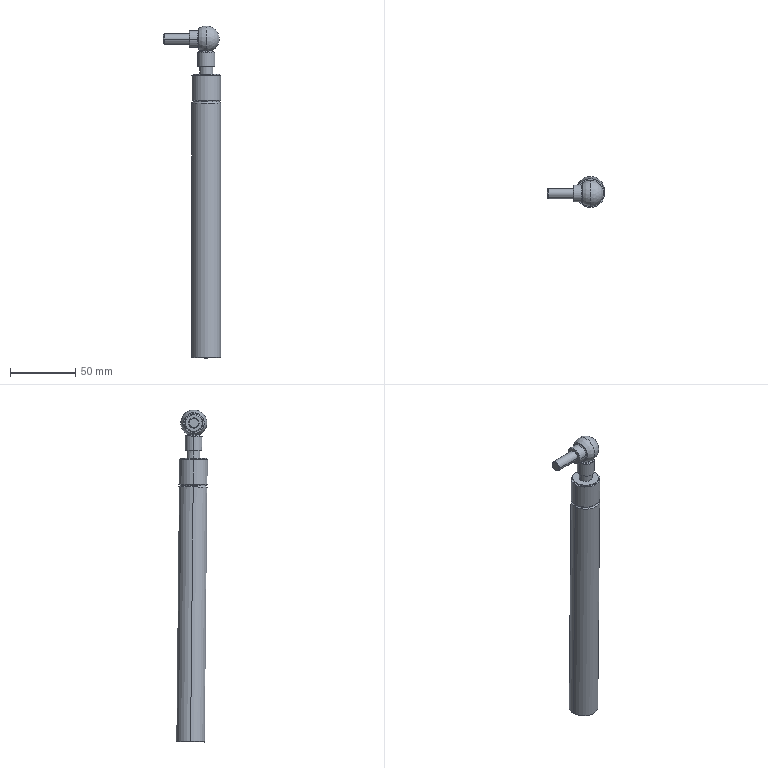Component | SolidWorks | GasSpringA-1 | 1 solid | 45 faces | box 44 x 24.24 x 255.09 mm | volume 50816 mm3 | cylinder 16 | cone 10 | plane 9 | torus 8 | sphere 2 | commonest cylinder face diameters 13 x4 22 x4 17 x2 8 x2 10 x2 20 x2
build123d program:
from build123d import *

# Parameters (mm, degrees)
SKETCH4_W           = 10.702
SKETCH4_H           = 20.307
CUT_EXTRUDE1_DEPTH  = 25
SKETCH5_R           = 6.5
BOSS_EXTRUDE1_DEPTH = 7
SKETCH6_R           = 4
BOSS_EXTRUDE2_DEPTH = 20
CHAMFER1_SIZE       = 0.5
CHAMFER2_SIZE       = 0.5
CHAMFER3_SIZE       = 0.2
SKETCH7_R           = 8.5
CUT_EXTRUDE2_DEPTH  = 600
FILLET1_R           = 1
SKETCH8_W           = 40.588
SKETCH8_H           = 852
CUT_EXTRUDE3_DEPTH  = 25
CHAMFER4_SIZE       = 0.5


with BuildPart() as part:
    # Sketch1 → Revolve1 (revolve)
    with BuildSketch(Plane.XY, mode=Mode.PRIVATE) as revolve1_sk:
        with BuildLine():
            Line((0, 0), (0, -680.998))
            ThreePointArc((0, -680.998), (-9.645, -673.639), (-5.095, -662.393))
            ThreePointArc((-5.095, -662.393), (-4.754, -661.55), (-5.477, -660.998))
            Line((-5.477, -660.998), (-6.5, -660.998))
            Line((-6.5, -660.998), (-6.5, -649.998))
            Line((-6.5, -649.998), (-5, -649.998))
            Line((-5, -649.998), (-5, -643.874))
            Line((-5, -643.874), (-10, -643.874))
            Line((-10, -643.874), (-10, -642.874))
            Line((-10, -642.874), (-11, -642.874))
            Line((-11, -642.874), (-11, -623.874))
            ThreePointArc((-11, -623.874), (-10, -622.874), (-11, -621.874))
            Line((-11, -621.874), (-11, 0))
            Line((-11, 0), (0, 0))
        make_face()
    revolve(revolve1_sk.sketch.rotate(Axis((0, 84.521, 0), (0, -1, 0)), 270), axis=Axis((0, 84.521, 0), (0, -1, 0)))

    # Sketch4 → Cut-Extrude1 (cut, symmetric)
    with BuildSketch(Plane(origin=(0, 0, 0), x_dir=(0, 0, -1), z_dir=(1, 0, 0))):
        with Locations((11.351, -671.855)):
            Rectangle(SKETCH4_W, SKETCH4_H)
    extrude(amount=CUT_EXTRUDE1_DEPTH, both=True, mode=Mode.SUBTRACT)

    # Sketch5 → Boss-Extrude1 (add)
    with BuildSketch(Plane(origin=(0, 0, -6), x_dir=(-1, 0, 0), z_dir=(0, 0, -1))):
        with Locations(Location((0, -670.998, 0), (0, 0, 180))):
            Circle(SKETCH5_R)
    extrude(amount=BOSS_EXTRUDE1_DEPTH)

    # Sketch6 → Boss-Extrude2 (add)
    with BuildSketch(Plane(origin=(0, 0, -13), x_dir=(-1, 0, 0), z_dir=(0, 0, -1))):
        with Locations((0, -670.998)):
            Circle(SKETCH6_R)
    extrude(amount=BOSS_EXTRUDE2_DEPTH)

    # Chamfer1
    chamfer1_edges = [part.edges().sort_by_distance(p)[0] for p in [
        (4, -670.998, -33),
    ]]
    chamfer(chamfer1_edges, length=CHAMFER1_SIZE)

    # Chamfer2
    chamfer2_edges = [part.edges().sort_by_distance(p)[0] for p in [
        (-6.5, -670.998, -6),
    ]]
    chamfer(chamfer2_edges, length=CHAMFER2_SIZE)

    # Chamfer3
    chamfer3_edges = [part.edges().sort_by_distance(p)[0] for p in [
        (-6.5, -670.998, -13),
    ]]
    chamfer(chamfer3_edges, length=CHAMFER3_SIZE)

    # Sketch7 → Cut-Extrude2 (cut)
    with BuildSketch(Plane(origin=(0, 0, 0), x_dir=(1, 0, 0), z_dir=(0, 1, 0))):
        with Locations(Location((0, 0, 0), (0, 0, 270))):
            Circle(SKETCH7_R)
    extrude(amount=-CUT_EXTRUDE2_DEPTH, mode=Mode.SUBTRACT)

    # Fillet1
    fillet1_edges = [part.edges().sort_by_distance(p)[0] for p in [
        (0, 0, -11),
    ]]
    fillet(fillet1_edges, radius=FILLET1_R)

    # Sketch8 → Cut-Extrude3 (cut, symmetric)
    with BuildSketch(Plane.XY):
        Rectangle(SKETCH8_W, SKETCH8_H)
    extrude(amount=CUT_EXTRUDE3_DEPTH, both=True, mode=Mode.SUBTRACT)

    # Chamfer4
    chamfer4_edges = [part.edges().sort_by_distance(p)[0] for p in [
        (0, -426, -11),
        (0, -426, -8.5),
    ]]
    chamfer(chamfer4_edges, length=CHAMFER4_SIZE)


solid = part.part

# Placed as in the assembly
solid = solid.moved(Location((899.814, -242.861, -680.808), (-89.408, 90, 0)))